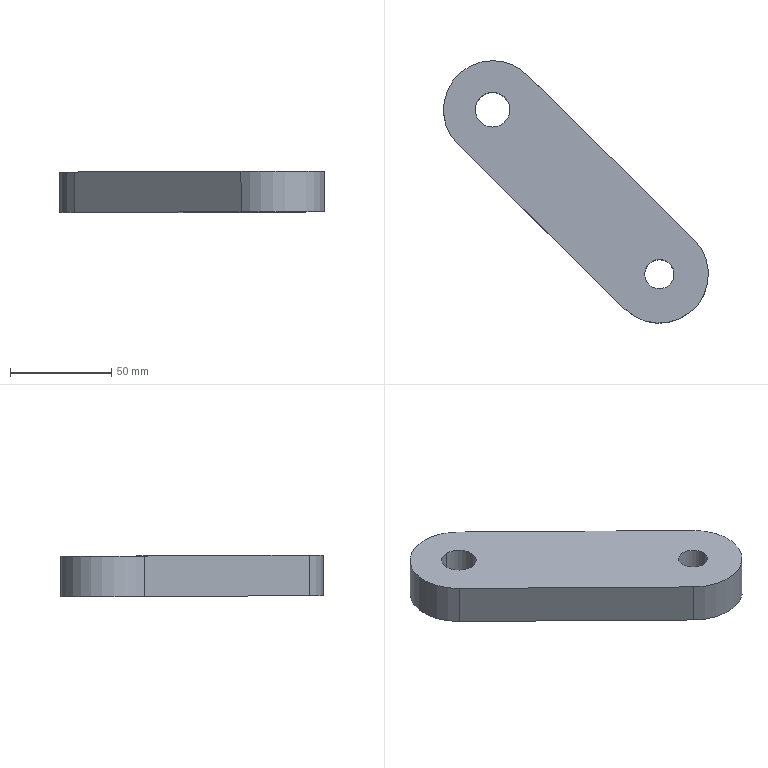Component | SolidWorks | RehabilitationChair-18-16-1 | 1 solid | 11 faces | box 131.13 x 130 x 20.52 mm | volume 141613 mm3 | cylinder 7 | plane 4 | commonest cylinder face diameters 48.527 x3 17.187 x2 14.46 x2
STEP:
#1=COLOUR_RGB('',0.7922,0.8196,0.9333);
#2=FILL_AREA_STYLE_COLOUR('',#1);
#3=FILL_AREA_STYLE('',(#2));
#4=SURFACE_STYLE_FILL_AREA(#3);
#5=SURFACE_SIDE_STYLE('',(#4));
#6=SURFACE_STYLE_USAGE(.BOTH.,#5);
#7=PRESENTATION_STYLE_ASSIGNMENT((#6));
#8=CARTESIAN_POINT('',(12.719,10.316,13.218));
#9=VERTEX_POINT('',#8);
#10=CARTESIAN_POINT('',(12.719,10.993,13.215));
#11=VERTEX_POINT('',#10);
#12=CARTESIAN_POINT('',(12.719,10.655,13.216));
#13=DIRECTION('',(-0.0003323,0.003798,1.));
#14=DIRECTION('',(0.,1.,-0.003798));
#15=AXIS2_PLACEMENT_3D('',#12,#13,#14);
#16=CIRCLE('',#15,0.3383);
#17=EDGE_CURVE('',#9,#11,#16,.T.);
#18=ORIENTED_EDGE('',*,*,#17,.T.);
#19=CARTESIAN_POINT('',(12.719,10.99,12.428));
#20=VERTEX_POINT('',#19);
#21=CARTESIAN_POINT('',(12.718,11.007,16.8));
#22=DIRECTION('',(0.0003323,-0.003798,-1.));
#23=VECTOR('',#22,39.37);
#24=LINE('',#21,#23);
#25=EDGE_CURVE('',#11,#20,#24,.T.);
#26=ORIENTED_EDGE('',*,*,#25,.T.);
#27=CARTESIAN_POINT('',(12.719,10.313,12.43));
#28=VERTEX_POINT('',#27);
#29=CARTESIAN_POINT('',(12.719,10.652,12.429));
#30=DIRECTION('',(-0.0003323,0.003798,1.));
#31=DIRECTION('',(0.,-1.,0.003798));
#32=AXIS2_PLACEMENT_3D('',#29,#30,#31);
#33=CIRCLE('',#32,0.3383);
#34=EDGE_CURVE('',#28,#20,#33,.T.);
#35=ORIENTED_EDGE('',*,*,#34,.F.);
#36=CARTESIAN_POINT('',(12.718,10.33,16.803));
#37=DIRECTION('',(0.0003323,-0.003798,-1.));
#38=VECTOR('',#37,39.37);
#39=LINE('',#36,#38);
#40=EDGE_CURVE('',#9,#28,#39,.T.);
#41=ORIENTED_EDGE('',*,*,#40,.F.);
#42=EDGE_LOOP('',(#18,#26,#35,#41));
#43=FACE_OUTER_BOUND('',#42,.T.);
#44=CARTESIAN_POINT('',(12.718,10.668,16.801));
#45=DIRECTION('',(0.0003323,-0.003798,-1.));
#46=DIRECTION('',(0.,-1.,0.003798));
#47=AXIS2_PLACEMENT_3D('',#44,#45,#46);
#48=CYLINDRICAL_SURFACE('',#47,0.3383);
#49=ADVANCED_FACE('',(#43),#48,.F.);
#50=CARTESIAN_POINT('',(15.971,7.162,12.443));
#51=VERTEX_POINT('',#50);
#52=CARTESIAN_POINT('',(15.971,7.732,12.441));
#53=VERTEX_POINT('',#52);
#54=CARTESIAN_POINT('',(15.971,7.447,12.442));
#55=DIRECTION('',(-0.0003323,0.003798,1.));
#56=DIRECTION('',(0.,1.,-0.003798));
#57=AXIS2_PLACEMENT_3D('',#54,#55,#56);
#58=CIRCLE('',#57,0.2846);
#59=EDGE_CURVE('',#51,#53,#58,.T.);
#60=ORIENTED_EDGE('',*,*,#59,.F.);
#61=CARTESIAN_POINT('',(15.971,7.165,13.231));
#62=VERTEX_POINT('',#61);
#63=CARTESIAN_POINT('',(15.971,7.162,12.422));
#64=DIRECTION('',(-0.0003323,0.003798,1.));
#65=VECTOR('',#64,39.37);
#66=LINE('',#63,#65);
#67=EDGE_CURVE('',#51,#62,#66,.T.);
#68=ORIENTED_EDGE('',*,*,#67,.T.);
#69=CARTESIAN_POINT('',(15.971,7.735,13.228));
#70=VERTEX_POINT('',#69);
#71=CARTESIAN_POINT('',(15.971,7.45,13.23));
#72=DIRECTION('',(-0.0003323,0.003798,1.));
#73=DIRECTION('',(0.,-1.,0.003798));
#74=AXIS2_PLACEMENT_3D('',#71,#72,#73);
#75=CIRCLE('',#74,0.2846);
#76=EDGE_CURVE('',#62,#70,#75,.T.);
#77=ORIENTED_EDGE('',*,*,#76,.T.);
#78=CARTESIAN_POINT('',(15.971,7.732,12.42));
#79=DIRECTION('',(-0.0003323,0.003798,1.));
#80=VECTOR('',#79,39.37);
#81=LINE('',#78,#80);
#82=EDGE_CURVE('',#53,#70,#81,.T.);
#83=ORIENTED_EDGE('',*,*,#82,.F.);
#84=EDGE_LOOP('',(#60,#68,#77,#83));
#85=FACE_OUTER_BOUND('',#84,.T.);
#86=CARTESIAN_POINT('',(15.971,7.447,12.421));
#87=DIRECTION('',(-0.0003323,0.003798,1.));
#88=DIRECTION('',(0.,1.,-0.003798));
#89=AXIS2_PLACEMENT_3D('',#86,#87,#88);
#90=CYLINDRICAL_SURFACE('',#89,0.2846);
#91=ADVANCED_FACE('',(#85),#90,.F.);
#92=CARTESIAN_POINT('',(13.39,11.332,12.427));
#93=VERTEX_POINT('',#92);
#94=CARTESIAN_POINT('',(12.719,11.607,12.425));
#95=VERTEX_POINT('',#94);
#96=CARTESIAN_POINT('',(12.719,10.652,12.429));
#97=DIRECTION('',(-0.0003323,0.003798,1.));
#98=DIRECTION('',(0.,-1.,0.003798));
#99=AXIS2_PLACEMENT_3D('',#96,#97,#98);
#100=CIRCLE('',#99,0.9553);
#101=EDGE_CURVE('',#93,#95,#100,.T.);
#102=ORIENTED_EDGE('',*,*,#101,.T.);
#103=CARTESIAN_POINT('',(12.719,11.61,13.213));
#104=VERTEX_POINT('',#103);
#105=CARTESIAN_POINT('',(12.719,11.607,12.425));
#106=DIRECTION('',(-0.0003323,0.003798,1.));
#107=VECTOR('',#106,39.37);
#108=LINE('',#105,#107);
#109=EDGE_CURVE('',#95,#104,#108,.T.);
#110=ORIENTED_EDGE('',*,*,#109,.T.);
#111=CARTESIAN_POINT('',(13.39,11.335,13.214));
#112=VERTEX_POINT('',#111);
#113=CARTESIAN_POINT('',(12.719,10.655,13.216));
#114=DIRECTION('',(-0.0003323,0.003798,1.));
#115=DIRECTION('',(0.,-1.,0.003798));
#116=AXIS2_PLACEMENT_3D('',#113,#114,#115);
#117=CIRCLE('',#116,0.9553);
#118=EDGE_CURVE('',#112,#104,#117,.T.);
#119=ORIENTED_EDGE('',*,*,#118,.F.);
#120=CARTESIAN_POINT('',(13.39,11.332,12.427));
#121=DIRECTION('',(-0.0003323,0.003798,1.));
#122=VECTOR('',#121,39.37);
#123=LINE('',#120,#122);
#124=EDGE_CURVE('',#93,#112,#123,.T.);
#125=ORIENTED_EDGE('',*,*,#124,.F.);
#126=EDGE_LOOP('',(#102,#110,#119,#125));
#127=FACE_OUTER_BOUND('',#126,.T.);
#128=CARTESIAN_POINT('',(12.719,10.652,12.429));
#129=DIRECTION('',(-0.0003323,0.003798,1.));
#130=DIRECTION('',(0.,1.,-0.003798));
#131=AXIS2_PLACEMENT_3D('',#128,#129,#130);
#132=CYLINDRICAL_SURFACE('',#131,0.9553);
#133=ADVANCED_FACE('',(#127),#132,.T.);
#134=ORIENTED_EDGE('',*,*,#25,.F.);
#135=CARTESIAN_POINT('',(12.719,10.655,13.216));
#136=DIRECTION('',(-0.0003323,0.003798,1.));
#137=DIRECTION('',(0.,1.,-0.003798));
#138=AXIS2_PLACEMENT_3D('',#135,#136,#137);
#139=CIRCLE('',#138,0.3383);
#140=EDGE_CURVE('',#11,#9,#139,.T.);
#141=ORIENTED_EDGE('',*,*,#140,.T.);
#142=ORIENTED_EDGE('',*,*,#40,.T.);
#143=CARTESIAN_POINT('',(12.719,10.652,12.429));
#144=DIRECTION('',(-0.0003323,0.003798,1.));
#145=DIRECTION('',(0.,-1.,0.003798));
#146=AXIS2_PLACEMENT_3D('',#143,#144,#145);
#147=CIRCLE('',#146,0.3383);
#148=EDGE_CURVE('',#20,#28,#147,.T.);
#149=ORIENTED_EDGE('',*,*,#148,.F.);
#150=EDGE_LOOP('',(#134,#141,#142,#149));
#151=FACE_OUTER_BOUND('',#150,.T.);
#152=CARTESIAN_POINT('',(12.718,10.668,16.801));
#153=DIRECTION('',(0.0003323,-0.003798,-1.));
#154=DIRECTION('',(0.,-1.,0.003798));
#155=AXIS2_PLACEMENT_3D('',#152,#153,#154);
#156=CYLINDRICAL_SURFACE('',#155,0.3383);
#157=ADVANCED_FACE('',(#151),#156,.F.);
#158=ORIENTED_EDGE('',*,*,#67,.F.);
#159=CARTESIAN_POINT('',(15.971,7.447,12.442));
#160=DIRECTION('',(-0.0003323,0.003798,1.));
#161=DIRECTION('',(0.,1.,-0.003798));
#162=AXIS2_PLACEMENT_3D('',#159,#160,#161);
#163=CIRCLE('',#162,0.2846);
#164=EDGE_CURVE('',#53,#51,#163,.T.);
#165=ORIENTED_EDGE('',*,*,#164,.F.);
#166=ORIENTED_EDGE('',*,*,#82,.T.);
#167=CARTESIAN_POINT('',(15.971,7.45,13.23));
#168=DIRECTION('',(-0.0003323,0.003798,1.));
#169=DIRECTION('',(0.,-1.,0.003798));
#170=AXIS2_PLACEMENT_3D('',#167,#168,#169);
#171=CIRCLE('',#170,0.2846);
#172=EDGE_CURVE('',#70,#62,#171,.T.);
#173=ORIENTED_EDGE('',*,*,#172,.T.);
#174=EDGE_LOOP('',(#158,#165,#166,#173));
#175=FACE_OUTER_BOUND('',#174,.T.);
#176=CARTESIAN_POINT('',(15.971,7.447,12.421));
#177=DIRECTION('',(-0.0003323,0.003798,1.));
#178=DIRECTION('',(0.,1.,-0.003798));
#179=AXIS2_PLACEMENT_3D('',#176,#177,#178);
#180=CYLINDRICAL_SURFACE('',#179,0.2846);
#181=ADVANCED_FACE('',(#175),#180,.F.);
#182=CARTESIAN_POINT('',(12.049,9.974,13.219));
#183=VERTEX_POINT('',#182);
#184=CARTESIAN_POINT('',(15.3,6.77,13.232));
#185=VERTEX_POINT('',#184);
#186=CARTESIAN_POINT('',(12.049,9.974,13.219));
#187=DIRECTION('',(0.7123,-0.7019,0.002903));
#188=VECTOR('',#187,39.37);
#189=LINE('',#186,#188);
#190=EDGE_CURVE('',#183,#185,#189,.T.);
#191=ORIENTED_EDGE('',*,*,#190,.F.);
#192=CARTESIAN_POINT('',(12.049,9.971,12.431));
#193=VERTEX_POINT('',#192);
#194=CARTESIAN_POINT('',(12.049,9.971,12.431));
#195=DIRECTION('',(-0.0003323,0.003798,1.));
#196=VECTOR('',#195,39.37);
#197=LINE('',#194,#196);
#198=EDGE_CURVE('',#193,#183,#197,.T.);
#199=ORIENTED_EDGE('',*,*,#198,.F.);
#200=CARTESIAN_POINT('',(15.301,6.767,12.445));
#201=VERTEX_POINT('',#200);
#202=CARTESIAN_POINT('',(12.049,9.971,12.431));
#203=DIRECTION('',(0.7123,-0.7019,0.002903));
#204=VECTOR('',#203,39.37);
#205=LINE('',#202,#204);
#206=EDGE_CURVE('',#193,#201,#205,.T.);
#207=ORIENTED_EDGE('',*,*,#206,.T.);
#208=CARTESIAN_POINT('',(15.301,6.767,12.445));
#209=DIRECTION('',(-0.0003323,0.003798,1.));
#210=VECTOR('',#209,39.37);
#211=LINE('',#208,#210);
#212=EDGE_CURVE('',#201,#185,#211,.T.);
#213=ORIENTED_EDGE('',*,*,#212,.T.);
#214=EDGE_LOOP('',(#191,#199,#207,#213));
#215=FACE_OUTER_BOUND('',#214,.T.);
#216=CARTESIAN_POINT('',(12.049,9.971,12.431));
#217=DIRECTION('',(0.7019,0.7123,-0.002472));
#218=DIRECTION('',(-0.7123,0.7019,0.));
#219=AXIS2_PLACEMENT_3D('',#216,#217,#218);
#220=PLANE('',#219);
#221=ADVANCED_FACE('',(#215),#220,.F.);
#222=ORIENTED_EDGE('',*,*,#109,.F.);
#223=CARTESIAN_POINT('',(12.719,10.652,12.429));
#224=DIRECTION('',(-0.0003323,0.003798,1.));
#225=DIRECTION('',(0.,-1.,0.003798));
#226=AXIS2_PLACEMENT_3D('',#223,#224,#225);
#227=CIRCLE('',#226,0.9553);
#228=EDGE_CURVE('',#95,#193,#227,.T.);
#229=ORIENTED_EDGE('',*,*,#228,.T.);
#230=ORIENTED_EDGE('',*,*,#198,.T.);
#231=CARTESIAN_POINT('',(12.719,10.655,13.216));
#232=DIRECTION('',(-0.0003323,0.003798,1.));
#233=DIRECTION('',(0.,-1.,0.003798));
#234=AXIS2_PLACEMENT_3D('',#231,#232,#233);
#235=CIRCLE('',#234,0.9553);
#236=EDGE_CURVE('',#104,#183,#235,.T.);
#237=ORIENTED_EDGE('',*,*,#236,.F.);
#238=EDGE_LOOP('',(#222,#229,#230,#237));
#239=FACE_OUTER_BOUND('',#238,.T.);
#240=CARTESIAN_POINT('',(12.719,10.652,12.429));
#241=DIRECTION('',(-0.0003323,0.003798,1.));
#242=DIRECTION('',(0.,1.,-0.003798));
#243=AXIS2_PLACEMENT_3D('',#240,#241,#242);
#244=CYLINDRICAL_SURFACE('',#243,0.9553);
#245=ADVANCED_FACE('',(#239),#244,.T.);
#246=CARTESIAN_POINT('',(16.641,8.13,13.227));
#247=VERTEX_POINT('',#246);
#248=CARTESIAN_POINT('',(15.971,7.45,13.23));
#249=DIRECTION('',(-0.0003323,0.003798,1.));
#250=DIRECTION('',(0.,-1.,0.003798));
#251=AXIS2_PLACEMENT_3D('',#248,#249,#250);
#252=CIRCLE('',#251,0.9553);
#253=EDGE_CURVE('',#185,#247,#252,.T.);
#254=ORIENTED_EDGE('',*,*,#253,.F.);
#255=ORIENTED_EDGE('',*,*,#212,.F.);
#256=CARTESIAN_POINT('',(16.642,8.127,12.44));
#257=VERTEX_POINT('',#256);
#258=CARTESIAN_POINT('',(15.971,7.447,12.442));
#259=DIRECTION('',(-0.0003323,0.003798,1.));
#260=DIRECTION('',(0.,-1.,0.003798));
#261=AXIS2_PLACEMENT_3D('',#258,#259,#260);
#262=CIRCLE('',#261,0.9553);
#263=EDGE_CURVE('',#201,#257,#262,.T.);
#264=ORIENTED_EDGE('',*,*,#263,.T.);
#265=CARTESIAN_POINT('',(16.642,8.127,12.44));
#266=DIRECTION('',(-0.0003323,0.003798,1.));
#267=VECTOR('',#266,39.37);
#268=LINE('',#265,#267);
#269=EDGE_CURVE('',#257,#247,#268,.T.);
#270=ORIENTED_EDGE('',*,*,#269,.T.);
#271=EDGE_LOOP('',(#254,#255,#264,#270));
#272=FACE_OUTER_BOUND('',#271,.T.);
#273=CARTESIAN_POINT('',(15.971,7.447,12.442));
#274=DIRECTION('',(-0.0003323,0.003798,1.));
#275=DIRECTION('',(0.,1.,-0.003798));
#276=AXIS2_PLACEMENT_3D('',#273,#274,#275);
#277=CYLINDRICAL_SURFACE('',#276,0.9553);
#278=ADVANCED_FACE('',(#272),#277,.T.);
#279=CARTESIAN_POINT('',(13.39,11.335,13.214));
#280=DIRECTION('',(-0.7123,0.7019,-0.002903));
#281=VECTOR('',#280,39.37);
#282=LINE('',#279,#281);
#283=EDGE_CURVE('',#247,#112,#282,.T.);
#284=ORIENTED_EDGE('',*,*,#283,.F.);
#285=ORIENTED_EDGE('',*,*,#269,.F.);
#286=CARTESIAN_POINT('',(13.39,11.332,12.427));
#287=DIRECTION('',(-0.7123,0.7019,-0.002903));
#288=VECTOR('',#287,39.37);
#289=LINE('',#286,#288);
#290=EDGE_CURVE('',#257,#93,#289,.T.);
#291=ORIENTED_EDGE('',*,*,#290,.T.);
#292=ORIENTED_EDGE('',*,*,#124,.T.);
#293=EDGE_LOOP('',(#284,#285,#291,#292));
#294=FACE_OUTER_BOUND('',#293,.T.);
#295=CARTESIAN_POINT('',(13.39,11.332,12.427));
#296=DIRECTION('',(-0.7019,-0.7123,0.002472));
#297=DIRECTION('',(0.7123,-0.7019,0.));
#298=AXIS2_PLACEMENT_3D('',#295,#296,#297);
#299=PLANE('',#298);
#300=ADVANCED_FACE('',(#294),#299,.F.);
#301=ORIENTED_EDGE('',*,*,#101,.F.);
#302=ORIENTED_EDGE('',*,*,#290,.F.);
#303=ORIENTED_EDGE('',*,*,#263,.F.);
#304=ORIENTED_EDGE('',*,*,#206,.F.);
#305=ORIENTED_EDGE('',*,*,#228,.F.);
#306=EDGE_LOOP('',(#301,#302,#303,#304,#305));
#307=FACE_OUTER_BOUND('',#306,.T.);
#308=ORIENTED_EDGE('',*,*,#34,.T.);
#309=ORIENTED_EDGE('',*,*,#148,.T.);
#310=EDGE_LOOP('',(#308,#309));
#311=FACE_BOUND('',#310,.T.);
#312=ORIENTED_EDGE('',*,*,#164,.T.);
#313=ORIENTED_EDGE('',*,*,#59,.T.);
#314=EDGE_LOOP('',(#312,#313));
#315=FACE_BOUND('',#314,.T.);
#316=CARTESIAN_POINT('',(12.719,10.652,12.429));
#317=DIRECTION('',(0.0003323,-0.003798,-1.));
#318=DIRECTION('',(0.,-1.,0.003798));
#319=AXIS2_PLACEMENT_3D('',#316,#317,#318);
#320=PLANE('',#319);
#321=ADVANCED_FACE('',(#307,#311,#315),#320,.T.);
#322=ORIENTED_EDGE('',*,*,#283,.T.);
#323=ORIENTED_EDGE('',*,*,#118,.T.);
#324=ORIENTED_EDGE('',*,*,#236,.T.);
#325=ORIENTED_EDGE('',*,*,#190,.T.);
#326=ORIENTED_EDGE('',*,*,#253,.T.);
#327=EDGE_LOOP('',(#322,#323,#324,#325,#326));
#328=FACE_OUTER_BOUND('',#327,.T.);
#329=ORIENTED_EDGE('',*,*,#172,.F.);
#330=ORIENTED_EDGE('',*,*,#76,.F.);
#331=EDGE_LOOP('',(#329,#330));
#332=FACE_BOUND('',#331,.T.);
#333=ORIENTED_EDGE('',*,*,#17,.F.);
#334=ORIENTED_EDGE('',*,*,#140,.F.);
#335=EDGE_LOOP('',(#333,#334));
#336=FACE_BOUND('',#335,.T.);
#337=CARTESIAN_POINT('',(12.719,10.655,13.216));
#338=DIRECTION('',(0.0003323,-0.003798,-1.));
#339=DIRECTION('',(0.,-1.,0.003798));
#340=AXIS2_PLACEMENT_3D('',#337,#338,#339);
#341=PLANE('',#340);
#342=ADVANCED_FACE('',(#328,#332,#336),#341,.F.);
#343=CLOSED_SHELL('',(#49,#91,#133,#157,#181,#221,#245,#278,#300,#321,#342));
#344=MANIFOLD_SOLID_BREP('',#343);
#345=STYLED_ITEM('',(#7),#344);
#346=(LENGTH_UNIT()NAMED_UNIT(*)SI_UNIT($,.METRE.));
#347=LENGTH_MEASURE_WITH_UNIT(LENGTH_MEASURE(0.0254),#346);
#348=DIMENSIONAL_EXPONENTS(1.,0.,0.,0.,0.,0.,0.);
#349=(CONVERSION_BASED_UNIT('',#347)LENGTH_UNIT()NAMED_UNIT(#348));
#350=UNCERTAINTY_MEASURE_WITH_UNIT(LENGTH_MEASURE(0.00001),#349,'','');
#351=(NAMED_UNIT(*)PLANE_ANGLE_UNIT()SI_UNIT($,.RADIAN.));
#352=(NAMED_UNIT(*)SI_UNIT($,.STERADIAN.)SOLID_ANGLE_UNIT());
#353=(GEOMETRIC_REPRESENTATION_CONTEXT(3)GLOBAL_UNCERTAINTY_ASSIGNED_CONTEXT((#350))GLOBAL_UNIT_ASSIGNED_CONTEXT((#349,#351,#352))REPRESENTATION_CONTEXT('',''));
#354=MECHANICAL_DESIGN_GEOMETRIC_PRESENTATION_REPRESENTATION('',(#345),#353);
#355=PRESENTATION_LAYER_ASSIGNMENT('','',(#345));
#356=CARTESIAN_POINT('',(0.,0.,0.));
#357=DIRECTION('',(0.,0.,1.));
#358=DIRECTION('',(1.,0.,0.));
#359=AXIS2_PLACEMENT_3D('',#356,#357,#358);
#360=(LENGTH_UNIT()NAMED_UNIT(*)SI_UNIT($,.METRE.));
#361=LENGTH_MEASURE_WITH_UNIT(LENGTH_MEASURE(0.0254),#360);
#362=DIMENSIONAL_EXPONENTS(1.,0.,0.,0.,0.,0.,0.);
#363=(CONVERSION_BASED_UNIT('',#361)LENGTH_UNIT()NAMED_UNIT(#362));
#364=UNCERTAINTY_MEASURE_WITH_UNIT(LENGTH_MEASURE(0.00001),#363,'','');
#365=(NAMED_UNIT(*)PLANE_ANGLE_UNIT()SI_UNIT($,.RADIAN.));
#366=(NAMED_UNIT(*)SI_UNIT($,.STERADIAN.)SOLID_ANGLE_UNIT());
#367=(GEOMETRIC_REPRESENTATION_CONTEXT(3)GLOBAL_UNCERTAINTY_ASSIGNED_CONTEXT((#364))GLOBAL_UNIT_ASSIGNED_CONTEXT((#363,#365,#366))REPRESENTATION_CONTEXT('',''));
#368=ADVANCED_BREP_SHAPE_REPRESENTATION('',(#344,#359),#367);